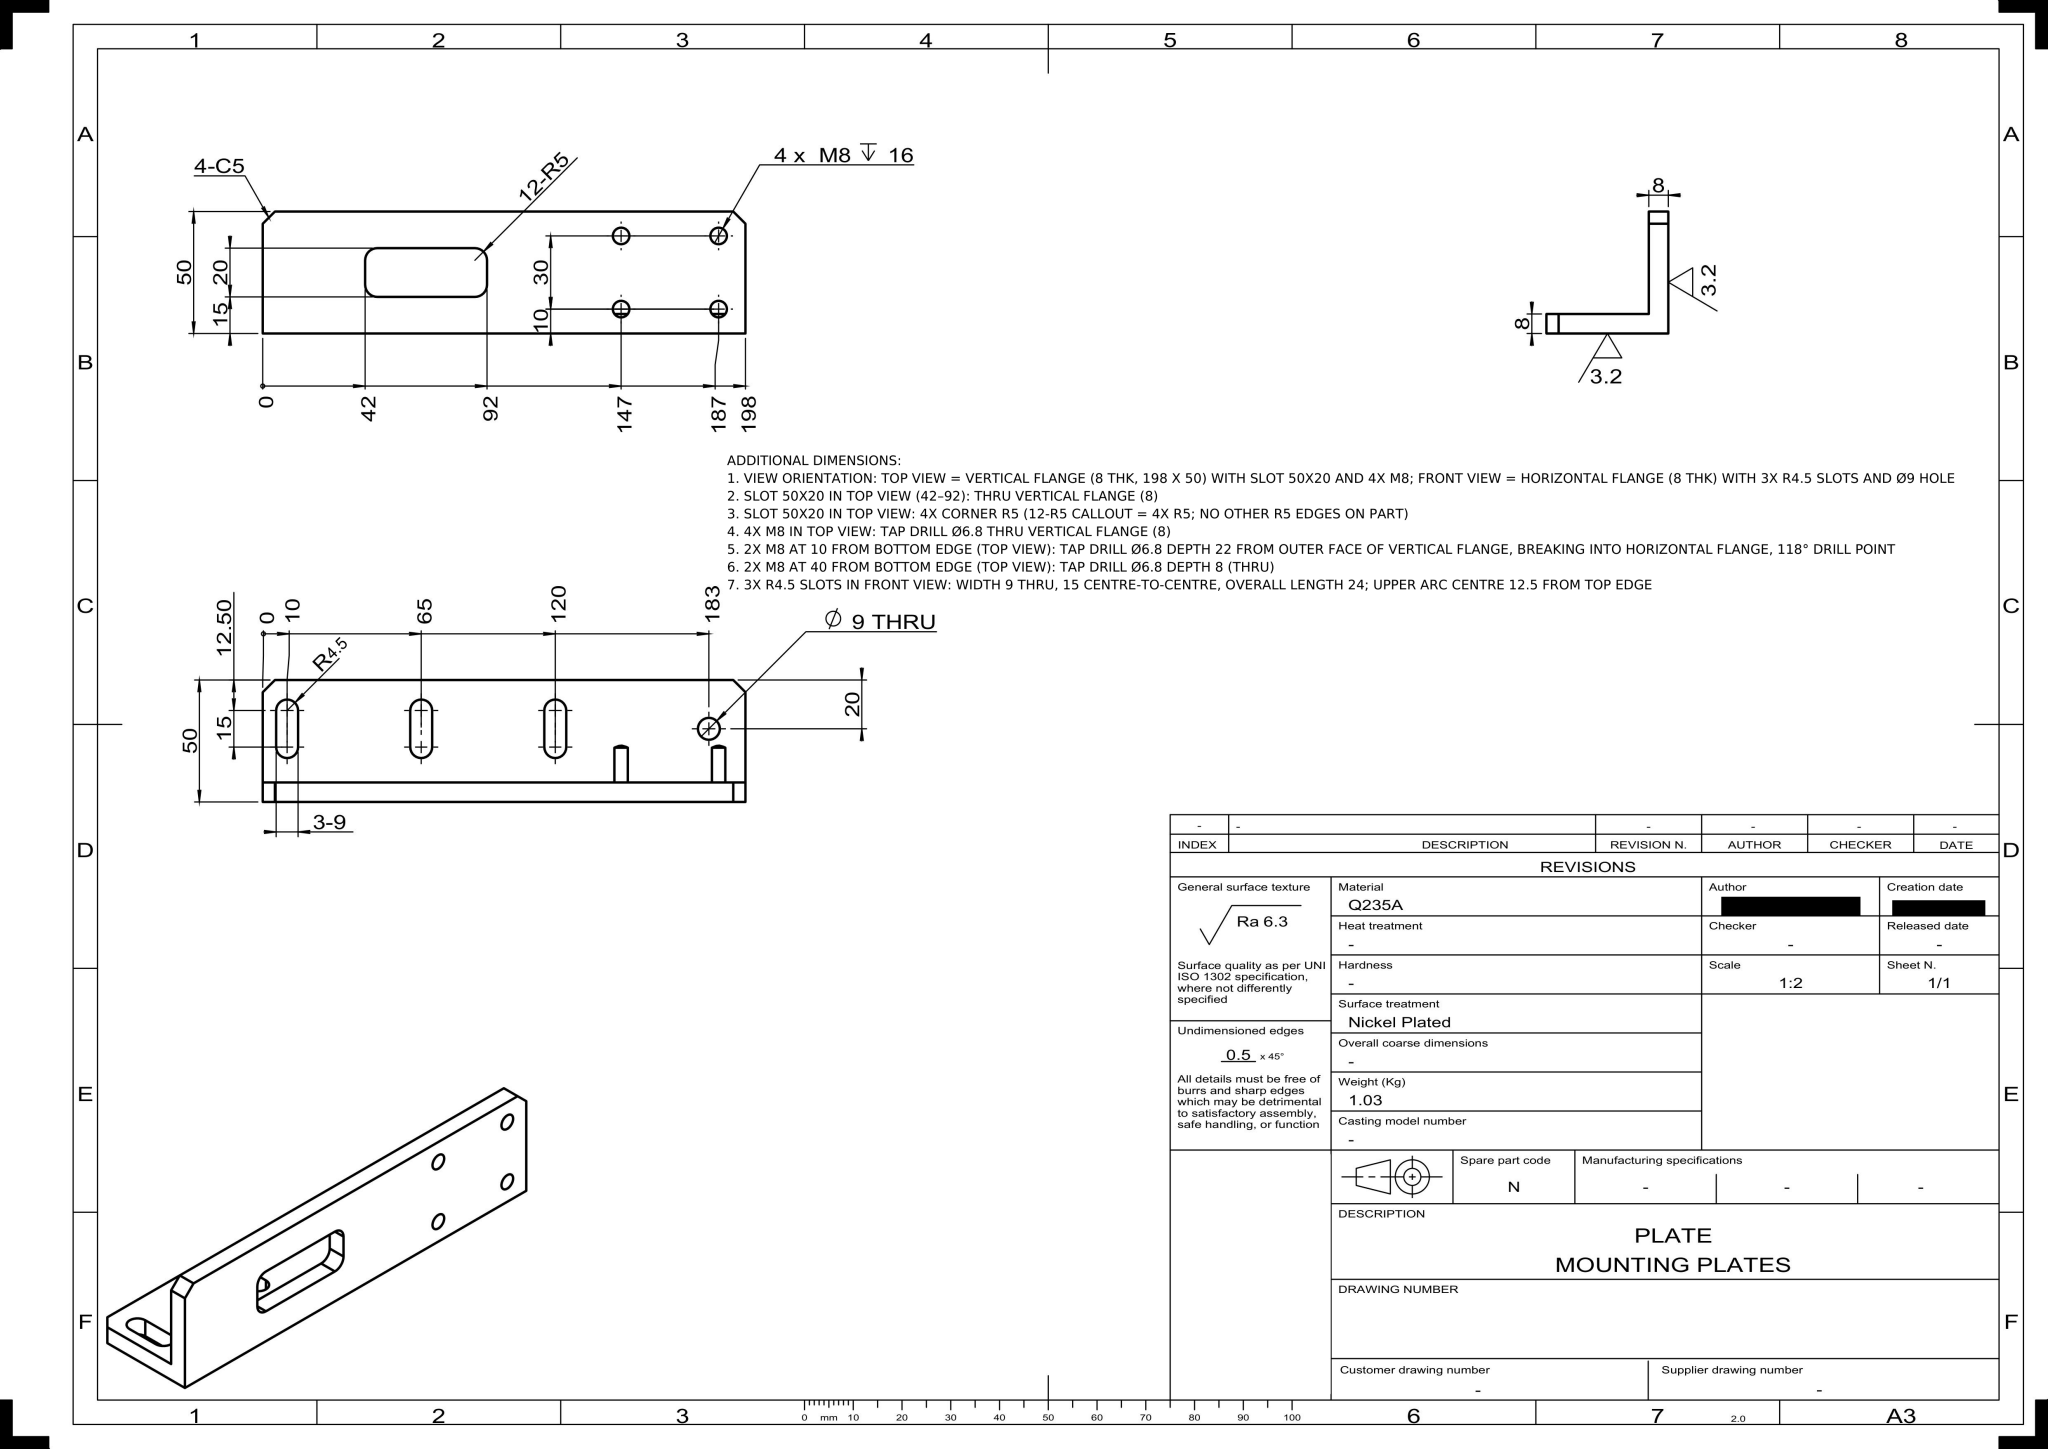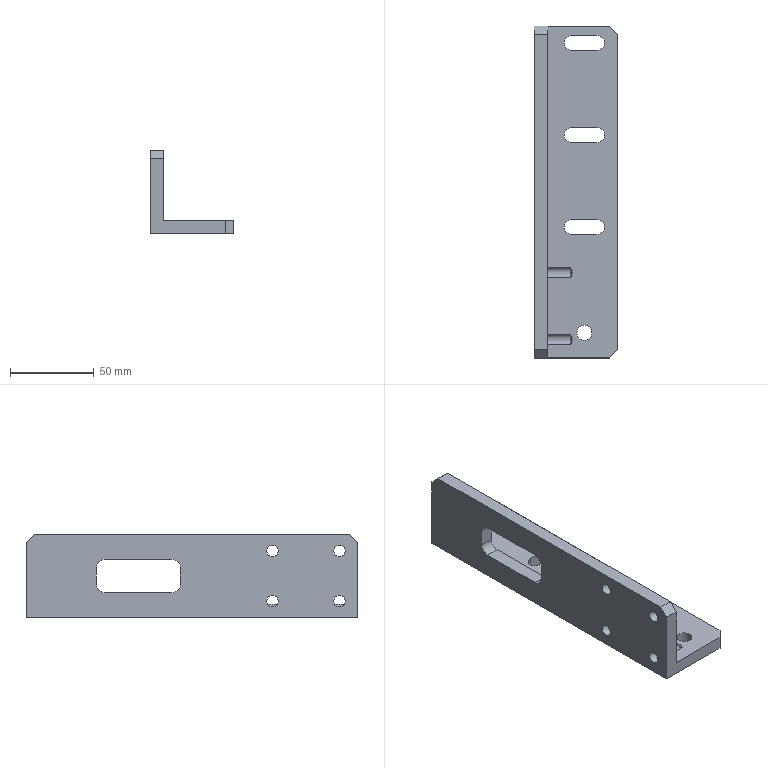Part | NX | mm | 1 solid | 39 faces | box 50 x 198 x 50 mm | volume 130907 mm3 | plane 22 | cylinder 15 | cone 2 | commonest cylinder face diameters 9 x7 6.8 x4 10 x4